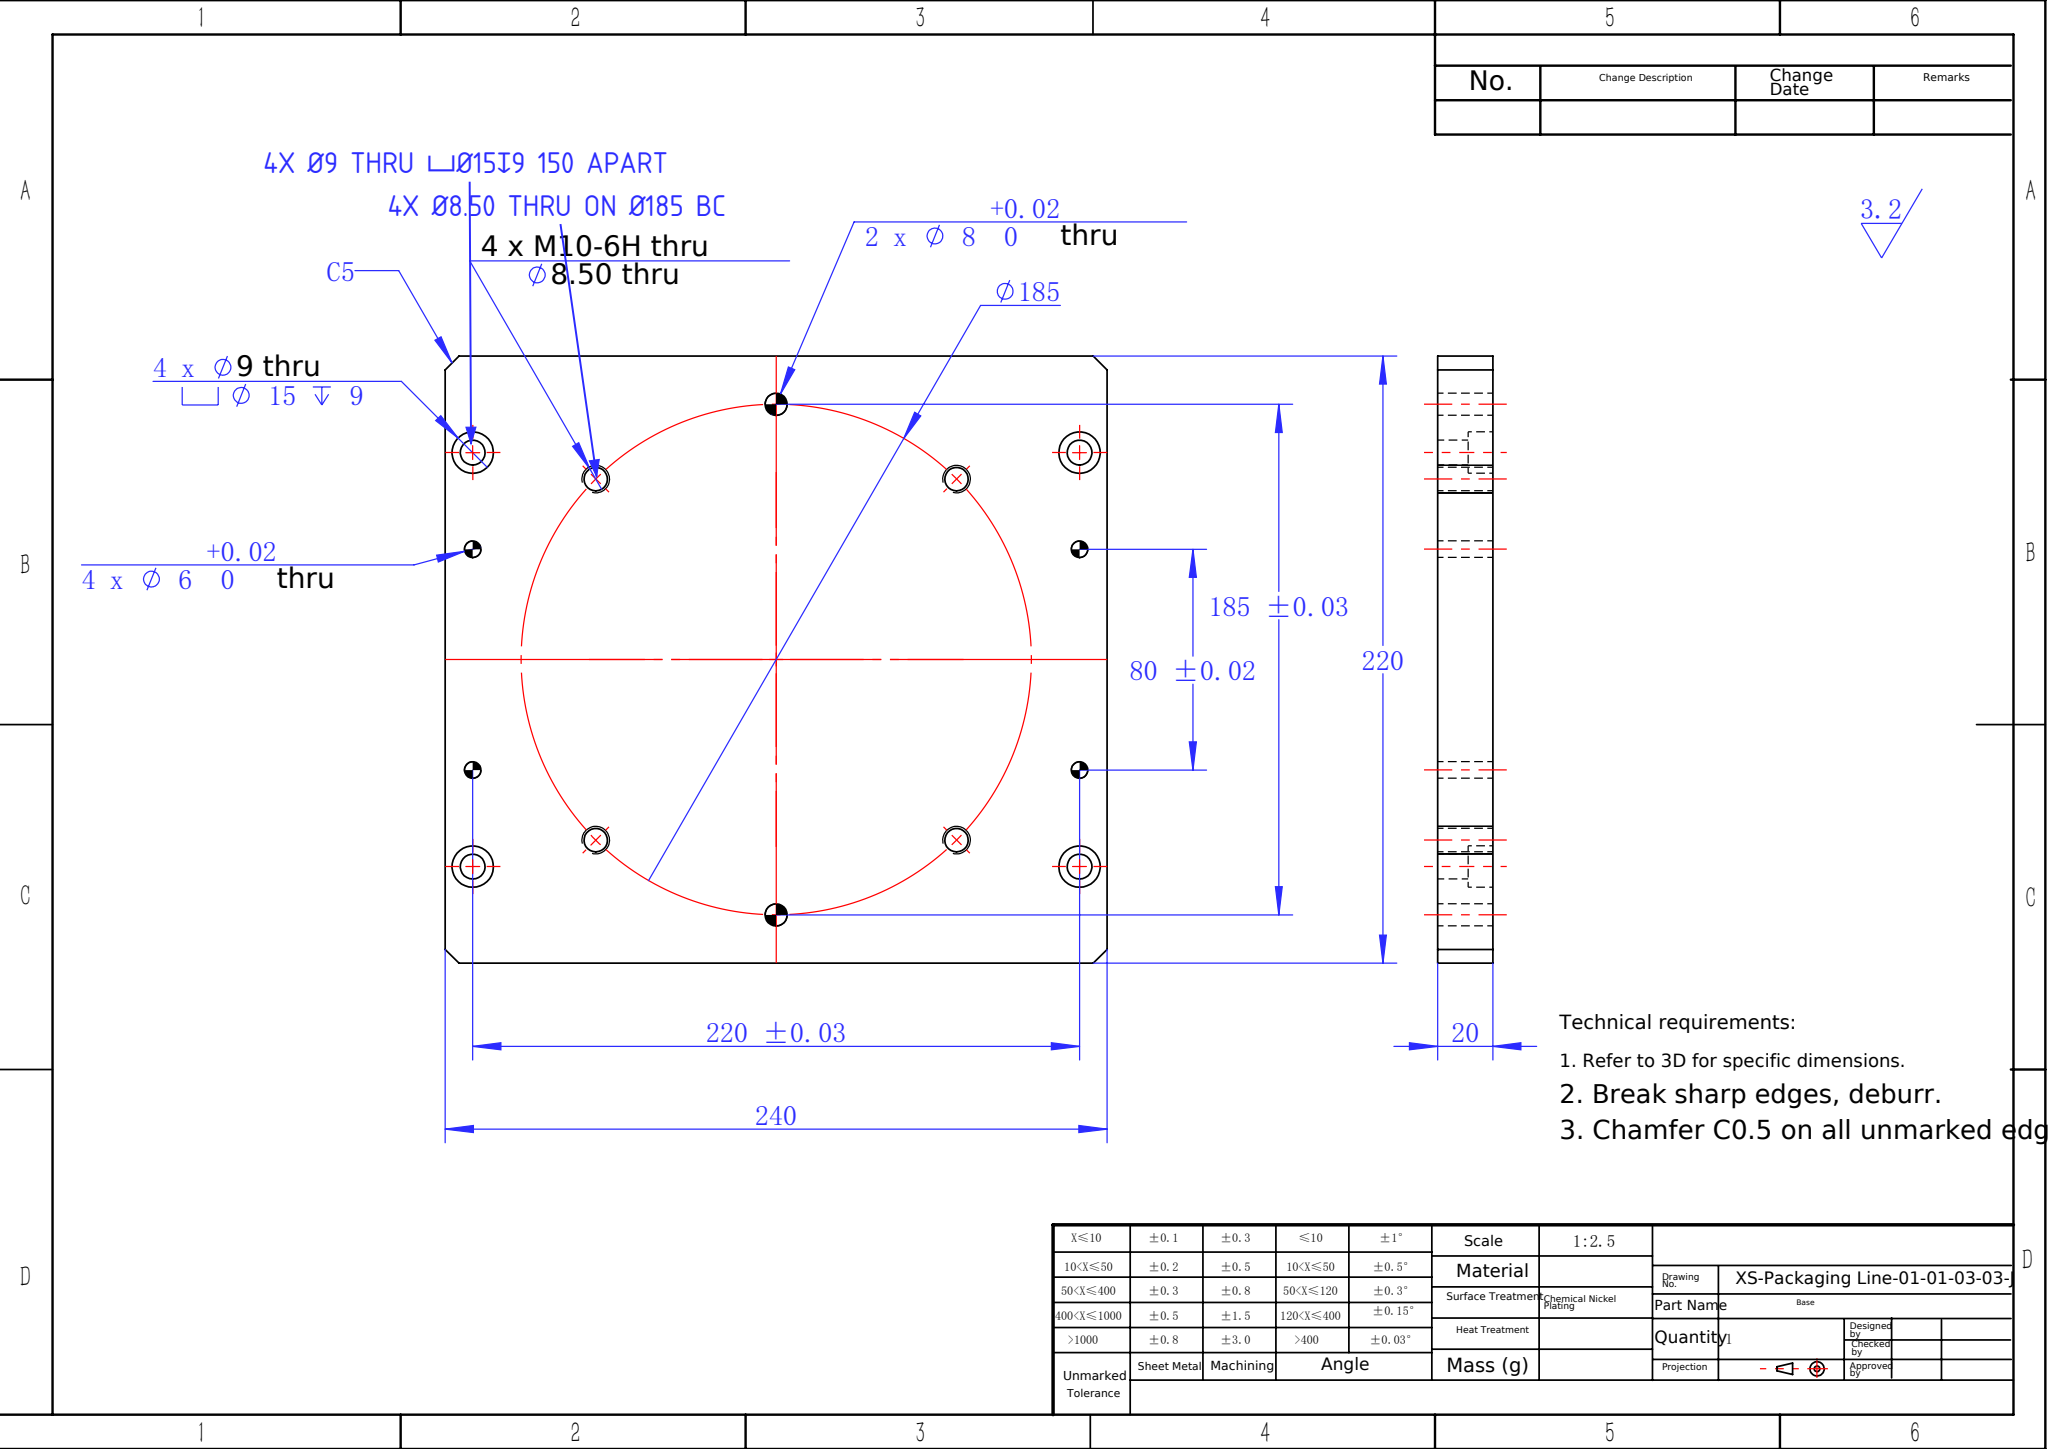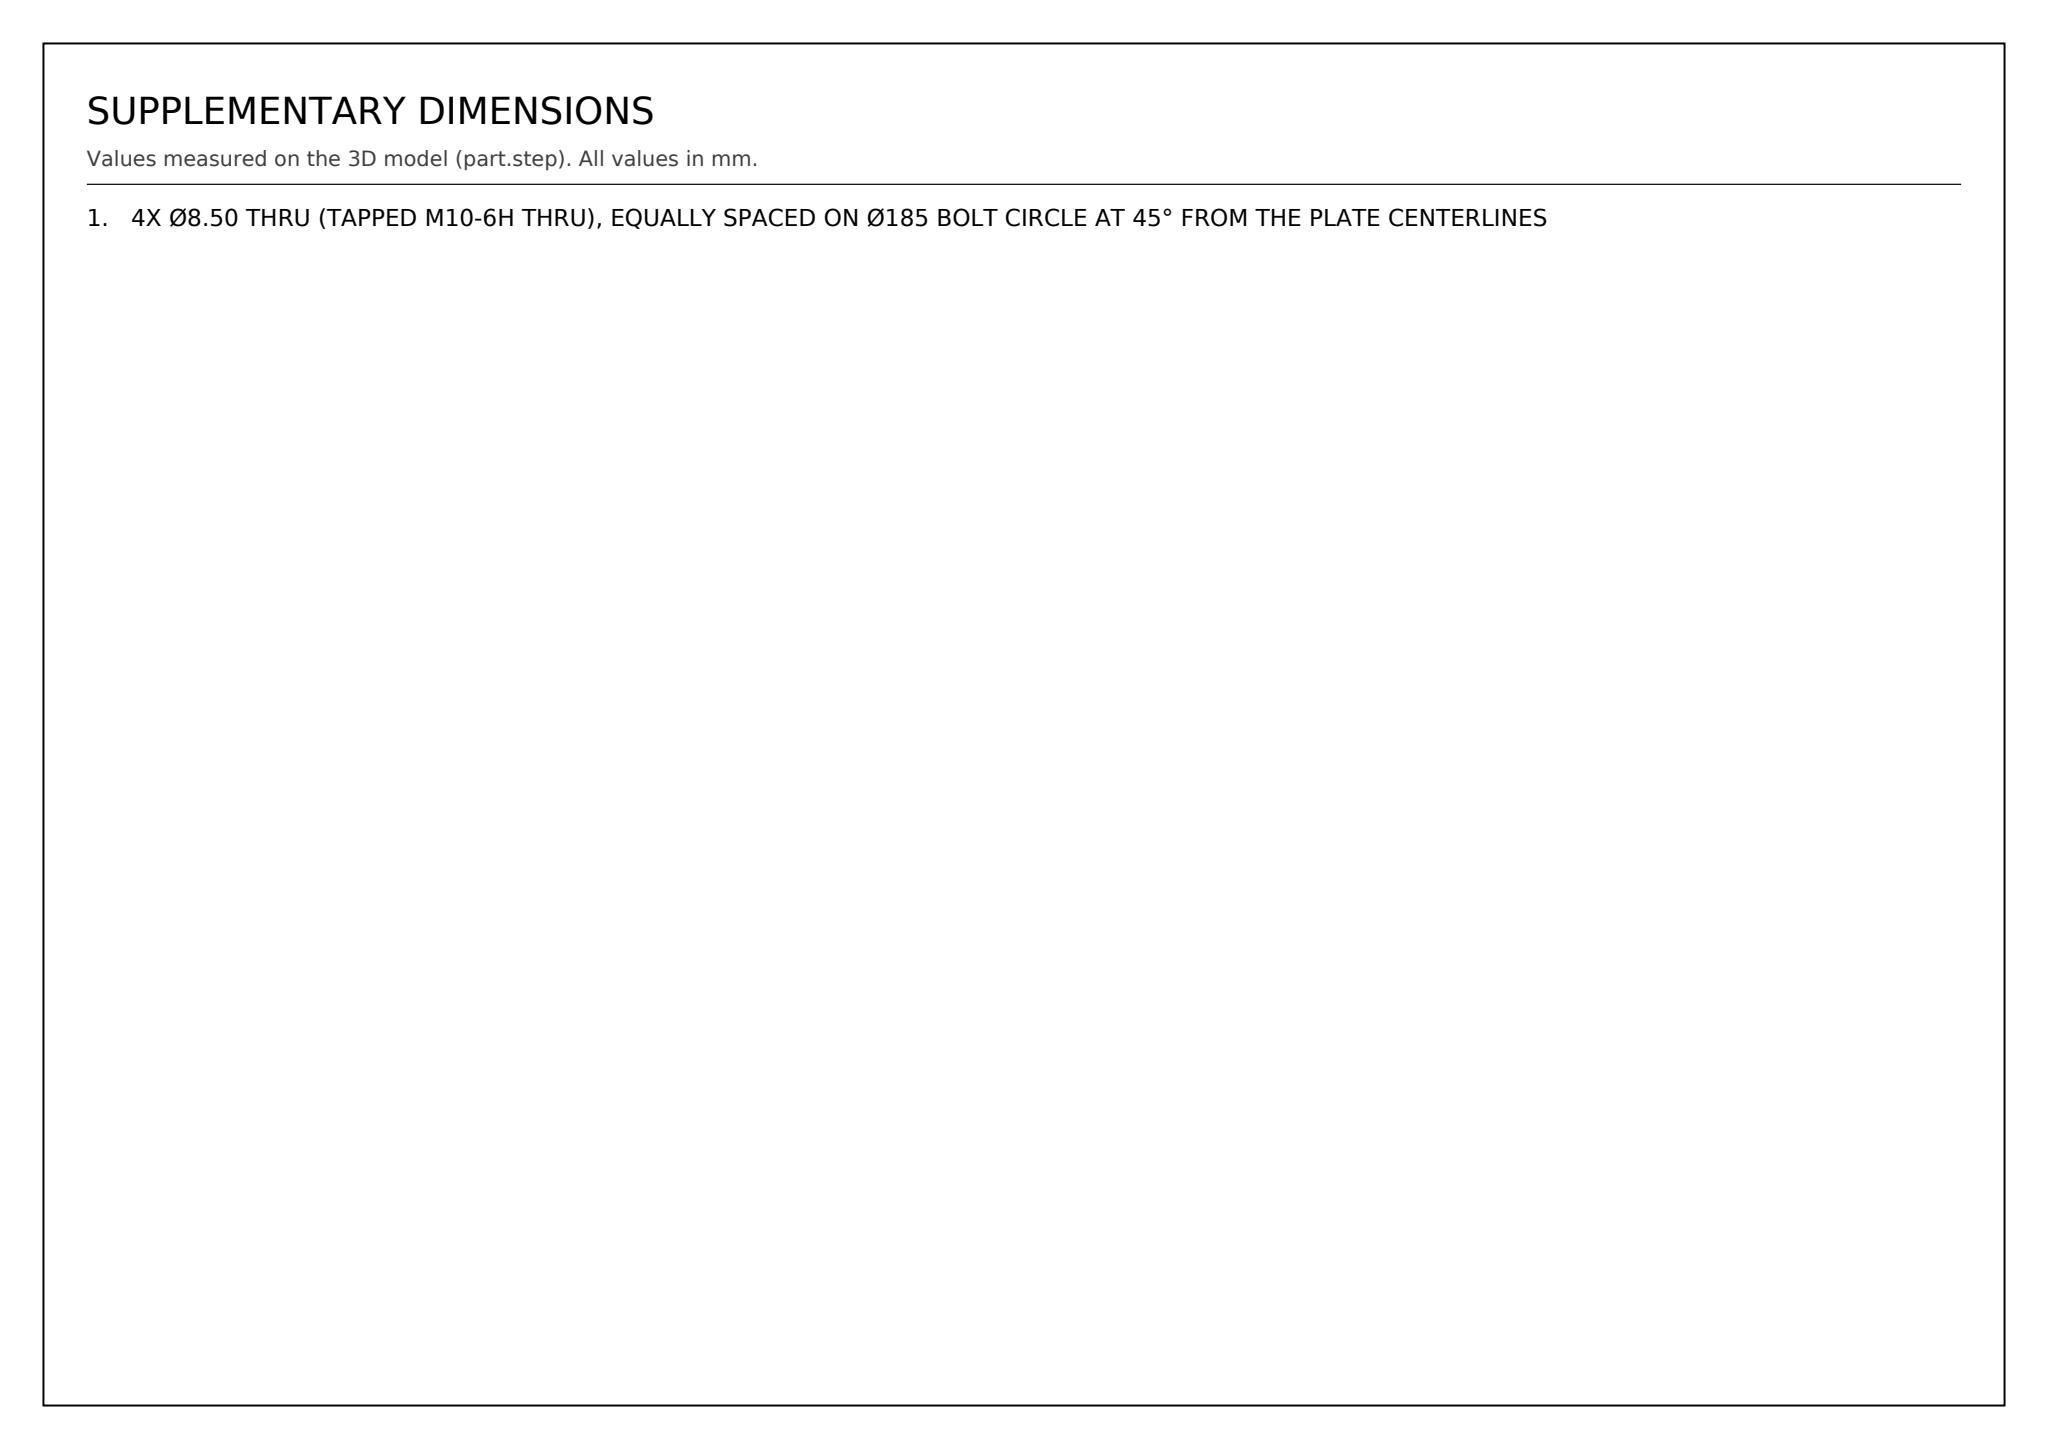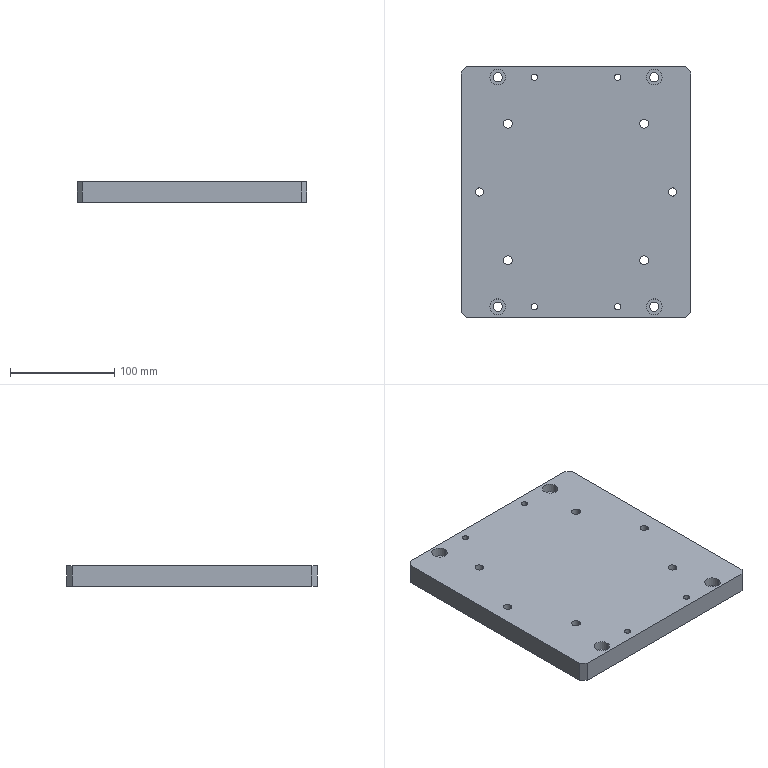Part | SolidWorks | mm | 1 solid | 50 faces | box 220 x 240 x 20 mm | volume 1037027 mm3 | cylinder 36 | plane 14 | commonest cylinder face diameters 8.5 x8 6 x8 15 x8 9 x8 8 x4
Drawing notes:
4 x Ø8.50 完全贯穿 (M10-6H 底孔), 位于 Ø185 B.C. @45° | from the solid: Four Ø8.0... actually Ø8.5 z-cylinders, L=20 (thru), at (44.59,54.59),(44.59,185.41),(175.41,54.59),(175.41,185.41); R=92.5 from plate center (110,120) = Ø185 B.C. at 45°
4X Ø9 THRU WITH Ø15 C'BORE DP 9: HOLE CENTERS 150 APART, EACH 35 FROM THE ADJACENT 220 EDGE (SYMMETRIC ABOUT PLATE CENTERLINE) | from the solid: cylinders dia 9.0 / dia 15.0 axis z at x = 35.0 and x = 185.0; bbox_xyz x = 220.0
4X Ø8.50 THRU (TAPPED M10-6H THRU), EQUALLY SPACED ON Ø185 BOLT CIRCLE AT 45° FROM THE PLATE CENTERLINES | from the solid: cylinders dia 8.5 axis z at (44.59,54.59), (44.59,185.41), (175.41,54.59), (175.41,185.41) = R92.5 about bbox center (110,120)
build123d program:
from build123d import *

# Parameters (mm, degrees)
SKETCH1_W                                       = 220
SKETCH1_H                                       = 240
BOSS_EXTRUDE1_DEPTH                             = 20
CHAMFER1_SIZE                                   = 5
M8_HEX_SOCKET_HEAD_CAP_SCREW_CBORE1_D           = 9
M8_HEX_SOCKET_HEAD_CAP_SCREW_CBORE1_CBORE_D     = 15
M8_HEX_SOCKET_HEAD_CAP_SCREW_CBORE1_CBORE_DEPTH = 9
F_6_0MM_DOWEL_PIN_HOLE1_D                       = 6
M10_TAPPED_HOLE1_D                              = 8.5
F_8_0MM_DOWEL_PIN_HOLE1_D                       = 8


with BuildPart() as part:
    # Sketch1 → Boss-Extrude1 (new body)
    with BuildSketch(Plane.XY):
        Rectangle(SKETCH1_W, SKETCH1_H)
    extrude(amount=BOSS_EXTRUDE1_DEPTH)

    # Chamfer1
    chamfer1_edges = [part.edges().sort_by_distance(p)[0] for p in [
        (110, -120, 10),
        (-110, -120, 10),
        (-110, 120, 10),
        (110, 120, 10),
    ]]
    chamfer(chamfer1_edges, length=CHAMFER1_SIZE)

    # M8 Hex Socket Head Cap Screw CBORE1 (through all)
    with Locations(Plane.XY.offset(20)):
        with Locations((75, 110), (-75, 110), (75, -110), (-75, -110)):
            CounterBoreHole(M8_HEX_SOCKET_HEAD_CAP_SCREW_CBORE1_D / 2, M8_HEX_SOCKET_HEAD_CAP_SCREW_CBORE1_CBORE_D / 2, M8_HEX_SOCKET_HEAD_CAP_SCREW_CBORE1_CBORE_DEPTH)

    # 6.0mm Dowel Pin Hole1 (through all)
    with Locations(Plane.XY.offset(20)):
        with Locations((40, 110), (-40, 110), (40, -110), (-40, -110)):
            Hole(F_6_0MM_DOWEL_PIN_HOLE1_D / 2)

    # M10 Tapped Hole1 (through all)
    with Locations(Plane.XY.offset(20)):
        with Locations((-65.407, -65.407), (-65.407, 65.407), (65.407, -65.407), (65.407, 65.407)):
            Hole(M10_TAPPED_HOLE1_D / 2)

    # 8.0mm Dowel Pin Hole1 (through all)
    with Locations(Plane.XY.offset(20)):
        with Locations((-92.5, 0), (92.5, 0)):
            Hole(F_8_0MM_DOWEL_PIN_HOLE1_D / 2)


solid = part.part